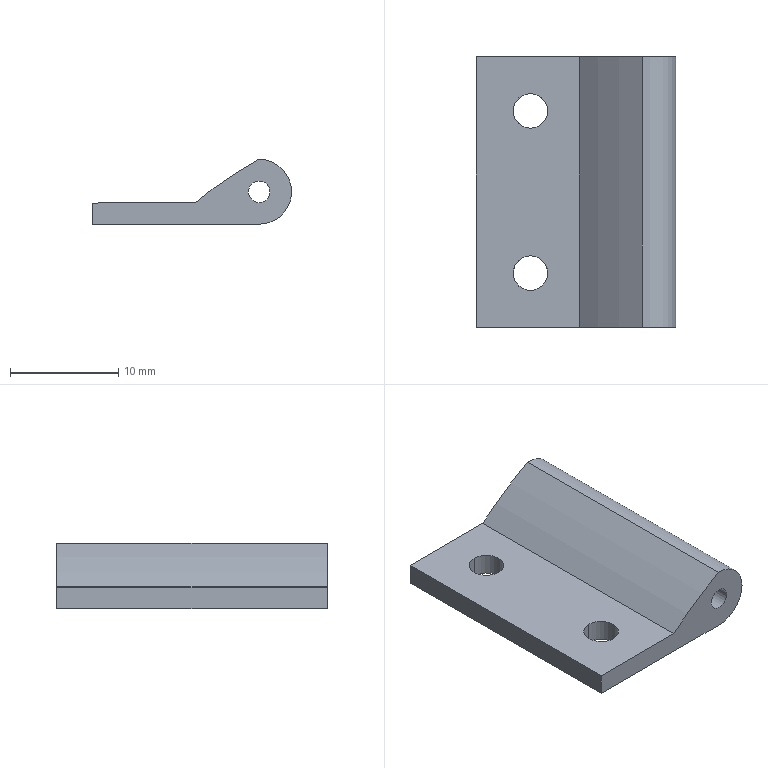Component | SolidWorks | CL201-M6-2-5 | 1 solid | 14 faces | box 18.43 x 25 x 6.04 mm | volume 1333 mm3 | cylinder 8 | plane 5 | spline 1 | commonest cylinder face diameters 3.2 x4 2 x2 6 x2
build123d program:
from build123d import *

# Parameters (mm, degrees)
SKETCH1_R           = 1
BOSS_EXTRUDE1_DEPTH = 25
SKETCH5_R           = 1.6
CUT_EXTRUDE3_DEPTH  = 48


with BuildPart() as part:
    # Sketch1 → Boss-Extrude1 (new body)
    with BuildSketch(Plane.XY):
        with BuildLine():
            Line((-63.314, 21.898), (-47.884, 21.898))
            Line((-47.884, 21.898), (-47.884, 19.898))
            Line((-47.884, 19.898), (-57.401, 19.898))
            add(Edge.make_bspline(
                [(-63.239, 15.899), (-59.863, 17.806), (-57.401, 19.898)],
                knots=[0, 0, 0, 0.7645, 0.7645, 0.7645], degree=2))
            ThreePointArc((-63.239, 15.899), (-66.314, 18.86), (-63.314, 21.898))
        make_face()
        with Locations((-63.314, 18.898)):
            Circle(SKETCH1_R, mode=Mode.SUBTRACT)
    extrude(amount=BOSS_EXTRUDE1_DEPTH)

    # Sketch5 → Cut-Extrude3 (cut)
    with BuildSketch(Plane.XZ.offset(-19.898)):
        with Locations(Location((-52.884, 20, 0), (0, 0, 270))):
            Circle(SKETCH5_R)
        with Locations(Location((-52.884, 5, 0), (0, 0, 270))):
            Circle(SKETCH5_R)
    extrude(amount=-CUT_EXTRUDE3_DEPTH, mode=Mode.SUBTRACT)


solid = part.part

# Placed as in the assembly
solid = solid.moved(Location((248.38, 1902.96, -163.788), (90, 0, -179.857)))
STEP:
#1=CARTESIAN_POINT('',(11.863,74.66,-7.305));
#2=VERTEX_POINT('',#1);
#3=CARTESIAN_POINT('',(11.863,74.786,-7.305));
#4=VERTEX_POINT('',#3);
#5=CARTESIAN_POINT('',(11.863,74.723,-7.305));
#6=DIRECTION('',(-0.002502,-0.,1.));
#7=DIRECTION('',(0.,1.,0.));
#8=AXIS2_PLACEMENT_3D('',#5,#6,#7);
#9=CIRCLE('',#8,0.06299);
#10=EDGE_CURVE('',#2,#4,#9,.T.);
#11=ORIENTED_EDGE('',*,*,#10,.F.);
#12=CARTESIAN_POINT('',(11.863,74.66,-7.227));
#13=VERTEX_POINT('',#12);
#14=CARTESIAN_POINT('',(11.867,74.66,-9.116));
#15=DIRECTION('',(-0.002502,-0.,1.));
#16=VECTOR('',#15,39.37);
#17=LINE('',#14,#16);
#18=EDGE_CURVE('',#2,#13,#17,.T.);
#19=ORIENTED_EDGE('',*,*,#18,.T.);
#20=CARTESIAN_POINT('',(11.863,74.786,-7.227));
#21=VERTEX_POINT('',#20);
#22=CARTESIAN_POINT('',(11.863,74.723,-7.227));
#23=DIRECTION('',(-0.002502,-0.,1.));
#24=DIRECTION('',(0.,1.,0.));
#25=AXIS2_PLACEMENT_3D('',#22,#23,#24);
#26=CIRCLE('',#25,0.06299);
#27=EDGE_CURVE('',#13,#21,#26,.T.);
#28=ORIENTED_EDGE('',*,*,#27,.T.);
#29=CARTESIAN_POINT('',(11.867,74.786,-9.116));
#30=DIRECTION('',(-0.002502,-0.,1.));
#31=VECTOR('',#30,39.37);
#32=LINE('',#29,#31);
#33=EDGE_CURVE('',#4,#21,#32,.T.);
#34=ORIENTED_EDGE('',*,*,#33,.F.);
#35=EDGE_LOOP('',(#11,#19,#28,#34));
#36=FACE_OUTER_BOUND('',#35,.T.);
#37=CARTESIAN_POINT('',(11.867,74.723,-9.116));
#38=DIRECTION('',(-0.002502,-0.,1.));
#39=DIRECTION('',(0.,1.,0.));
#40=AXIS2_PLACEMENT_3D('',#37,#38,#39);
#41=CYLINDRICAL_SURFACE('',#40,0.06299);
#42=ADVANCED_FACE('',(#36),#41,.F.);
#43=CARTESIAN_POINT('',(11.863,74.069,-7.305));
#44=VERTEX_POINT('',#43);
#45=CARTESIAN_POINT('',(11.863,74.195,-7.305));
#46=VERTEX_POINT('',#45);
#47=CARTESIAN_POINT('',(11.863,74.132,-7.305));
#48=DIRECTION('',(-0.002502,-0.,1.));
#49=DIRECTION('',(0.,1.,0.));
#50=AXIS2_PLACEMENT_3D('',#47,#48,#49);
#51=CIRCLE('',#50,0.06299);
#52=EDGE_CURVE('',#44,#46,#51,.T.);
#53=ORIENTED_EDGE('',*,*,#52,.F.);
#54=CARTESIAN_POINT('',(11.863,74.069,-7.227));
#55=VERTEX_POINT('',#54);
#56=CARTESIAN_POINT('',(11.867,74.069,-9.116));
#57=DIRECTION('',(-0.002502,-0.,1.));
#58=VECTOR('',#57,39.37);
#59=LINE('',#56,#58);
#60=EDGE_CURVE('',#44,#55,#59,.T.);
#61=ORIENTED_EDGE('',*,*,#60,.T.);
#62=CARTESIAN_POINT('',(11.863,74.195,-7.227));
#63=VERTEX_POINT('',#62);
#64=CARTESIAN_POINT('',(11.863,74.132,-7.227));
#65=DIRECTION('',(-0.002502,-0.,1.));
#66=DIRECTION('',(0.,1.,0.));
#67=AXIS2_PLACEMENT_3D('',#64,#65,#66);
#68=CIRCLE('',#67,0.06299);
#69=EDGE_CURVE('',#55,#63,#68,.T.);
#70=ORIENTED_EDGE('',*,*,#69,.T.);
#71=CARTESIAN_POINT('',(11.867,74.195,-9.116));
#72=DIRECTION('',(-0.002502,-0.,1.));
#73=VECTOR('',#72,39.37);
#74=LINE('',#71,#73);
#75=EDGE_CURVE('',#46,#63,#74,.T.);
#76=ORIENTED_EDGE('',*,*,#75,.F.);
#77=EDGE_LOOP('',(#53,#61,#70,#76));
#78=FACE_OUTER_BOUND('',#77,.T.);
#79=CARTESIAN_POINT('',(11.867,74.132,-9.116));
#80=DIRECTION('',(-0.002502,-0.,1.));
#81=DIRECTION('',(0.,1.,0.));
#82=AXIS2_PLACEMENT_3D('',#79,#80,#81);
#83=CYLINDRICAL_SURFACE('',#82,0.06299);
#84=ADVANCED_FACE('',(#78),#83,.F.);
#85=CARTESIAN_POINT('',(12.313,73.935,-7.186));
#86=VERTEX_POINT('',#85);
#87=CARTESIAN_POINT('',(12.234,73.935,-7.186));
#88=VERTEX_POINT('',#87);
#89=CARTESIAN_POINT('',(12.273,73.935,-7.186));
#90=DIRECTION('',(0.,-1.,-0.));
#91=DIRECTION('',(-1.,0.,-0.002502));
#92=AXIS2_PLACEMENT_3D('',#89,#90,#91);
#93=CIRCLE('',#92,0.03937);
#94=EDGE_CURVE('',#86,#88,#93,.T.);
#95=ORIENTED_EDGE('',*,*,#94,.T.);
#96=CARTESIAN_POINT('',(12.234,74.92,-7.186));
#97=VERTEX_POINT('',#96);
#98=CARTESIAN_POINT('',(12.234,73.935,-7.186));
#99=DIRECTION('',(-0.,1.,0.));
#100=VECTOR('',#99,39.37);
#101=LINE('',#98,#100);
#102=EDGE_CURVE('',#88,#97,#101,.T.);
#103=ORIENTED_EDGE('',*,*,#102,.T.);
#104=CARTESIAN_POINT('',(12.313,74.92,-7.186));
#105=VERTEX_POINT('',#104);
#106=CARTESIAN_POINT('',(12.273,74.92,-7.186));
#107=DIRECTION('',(0.,-1.,-0.));
#108=DIRECTION('',(-1.,0.,-0.002502));
#109=AXIS2_PLACEMENT_3D('',#106,#107,#108);
#110=CIRCLE('',#109,0.03937);
#111=EDGE_CURVE('',#105,#97,#110,.T.);
#112=ORIENTED_EDGE('',*,*,#111,.F.);
#113=CARTESIAN_POINT('',(12.313,73.935,-7.186));
#114=DIRECTION('',(-0.,1.,0.));
#115=VECTOR('',#114,39.37);
#116=LINE('',#113,#115);
#117=EDGE_CURVE('',#86,#105,#116,.T.);
#118=ORIENTED_EDGE('',*,*,#117,.F.);
#119=EDGE_LOOP('',(#95,#103,#112,#118));
#120=FACE_OUTER_BOUND('',#119,.T.);
#121=CARTESIAN_POINT('',(12.273,73.935,-7.186));
#122=DIRECTION('',(-0.,1.,0.));
#123=DIRECTION('',(1.,0.,0.002502));
#124=AXIS2_PLACEMENT_3D('',#121,#122,#123);
#125=CYLINDRICAL_SURFACE('',#124,0.03937);
#126=ADVANCED_FACE('',(#120),#125,.F.);
#127=CARTESIAN_POINT('',(12.391,73.935,-7.186));
#128=VERTEX_POINT('',#127);
#129=CARTESIAN_POINT('',(12.27,73.935,-7.068));
#130=VERTEX_POINT('',#129);
#131=CARTESIAN_POINT('',(12.273,73.935,-7.186));
#132=DIRECTION('',(0.,-1.,-0.));
#133=DIRECTION('',(-1.,0.,-0.002502));
#134=AXIS2_PLACEMENT_3D('',#131,#132,#133);
#135=CIRCLE('',#134,0.1181);
#136=EDGE_CURVE('',#128,#130,#135,.T.);
#137=ORIENTED_EDGE('',*,*,#136,.F.);
#138=CARTESIAN_POINT('',(12.391,74.92,-7.186));
#139=VERTEX_POINT('',#138);
#140=CARTESIAN_POINT('',(12.391,73.935,-7.186));
#141=DIRECTION('',(-0.,1.,0.));
#142=VECTOR('',#141,39.37);
#143=LINE('',#140,#142);
#144=EDGE_CURVE('',#128,#139,#143,.T.);
#145=ORIENTED_EDGE('',*,*,#144,.T.);
#146=CARTESIAN_POINT('',(12.27,74.92,-7.068));
#147=VERTEX_POINT('',#146);
#148=CARTESIAN_POINT('',(12.273,74.92,-7.186));
#149=DIRECTION('',(0.,-1.,-0.));
#150=DIRECTION('',(-1.,0.,-0.002502));
#151=AXIS2_PLACEMENT_3D('',#148,#149,#150);
#152=CIRCLE('',#151,0.1181);
#153=EDGE_CURVE('',#139,#147,#152,.T.);
#154=ORIENTED_EDGE('',*,*,#153,.T.);
#155=CARTESIAN_POINT('',(12.27,73.935,-7.068));
#156=DIRECTION('',(-0.,1.,0.));
#157=VECTOR('',#156,39.37);
#158=LINE('',#155,#157);
#159=EDGE_CURVE('',#130,#147,#158,.T.);
#160=ORIENTED_EDGE('',*,*,#159,.F.);
#161=EDGE_LOOP('',(#137,#145,#154,#160));
#162=FACE_OUTER_BOUND('',#161,.T.);
#163=CARTESIAN_POINT('',(12.273,73.935,-7.186));
#164=DIRECTION('',(-0.,1.,0.));
#165=DIRECTION('',(1.,0.,0.002502));
#166=AXIS2_PLACEMENT_3D('',#163,#164,#165);
#167=CYLINDRICAL_SURFACE('',#166,0.1181);
#168=ADVANCED_FACE('',(#162),#167,.T.);
#169=CARTESIAN_POINT('',(12.041,73.935,-7.226));
#170=VERTEX_POINT('',#169);
#171=CARTESIAN_POINT('',(12.27,73.935,-7.068));
#172=CARTESIAN_POINT('',(12.137,73.935,-7.143));
#173=CARTESIAN_POINT('',(12.041,73.935,-7.226));
#174=B_SPLINE_CURVE_WITH_KNOTS('',2,(#171,#172,#173),.UNSPECIFIED.,.F.,.F.,(3,3),(0.,0.7645),.UNSPECIFIED.);
#175=EDGE_CURVE('',#130,#170,#174,.T.);
#176=ORIENTED_EDGE('',*,*,#175,.T.);
#177=CARTESIAN_POINT('',(11.666,73.935,-7.227));
#178=VERTEX_POINT('',#177);
#179=CARTESIAN_POINT('',(12.041,73.935,-7.226));
#180=DIRECTION('',(-1.,-0.,-0.002502));
#181=VECTOR('',#180,39.37);
#182=LINE('',#179,#181);
#183=EDGE_CURVE('',#170,#178,#182,.T.);
#184=ORIENTED_EDGE('',*,*,#183,.T.);
#185=CARTESIAN_POINT('',(11.666,73.935,-7.306));
#186=VERTEX_POINT('',#185);
#187=CARTESIAN_POINT('',(11.666,73.935,-7.306));
#188=DIRECTION('',(0.002502,0.,-1.));
#189=VECTOR('',#188,39.37);
#190=LINE('',#187,#189);
#191=EDGE_CURVE('',#178,#186,#190,.T.);
#192=ORIENTED_EDGE('',*,*,#191,.T.);
#193=CARTESIAN_POINT('',(12.274,73.935,-7.304));
#194=VERTEX_POINT('',#193);
#195=CARTESIAN_POINT('',(12.274,73.935,-7.304));
#196=DIRECTION('',(1.,0.,0.002502));
#197=VECTOR('',#196,39.37);
#198=LINE('',#195,#197);
#199=EDGE_CURVE('',#186,#194,#198,.T.);
#200=ORIENTED_EDGE('',*,*,#199,.T.);
#201=CARTESIAN_POINT('',(12.273,73.935,-7.186));
#202=DIRECTION('',(0.,-1.,-0.));
#203=DIRECTION('',(-1.,0.,-0.002502));
#204=AXIS2_PLACEMENT_3D('',#201,#202,#203);
#205=CIRCLE('',#204,0.1181);
#206=EDGE_CURVE('',#194,#128,#205,.T.);
#207=ORIENTED_EDGE('',*,*,#206,.T.);
#208=ORIENTED_EDGE('',*,*,#136,.T.);
#209=EDGE_LOOP('',(#176,#184,#192,#200,#207,#208));
#210=FACE_OUTER_BOUND('',#209,.T.);
#211=ORIENTED_EDGE('',*,*,#94,.F.);
#212=CARTESIAN_POINT('',(12.273,73.935,-7.186));
#213=DIRECTION('',(0.,-1.,-0.));
#214=DIRECTION('',(-1.,0.,-0.002502));
#215=AXIS2_PLACEMENT_3D('',#212,#213,#214);
#216=CIRCLE('',#215,0.03937);
#217=EDGE_CURVE('',#88,#86,#216,.T.);
#218=ORIENTED_EDGE('',*,*,#217,.F.);
#219=EDGE_LOOP('',(#211,#218));
#220=FACE_BOUND('',#219,.T.);
#221=CARTESIAN_POINT('',(12.146,73.935,-7.145));
#222=DIRECTION('',(-0.,1.,0.));
#223=DIRECTION('',(1.,0.,0.002502));
#224=AXIS2_PLACEMENT_3D('',#221,#222,#223);
#225=PLANE('',#224);
#226=ADVANCED_FACE('',(#210,#220),#225,.F.);
#227=CARTESIAN_POINT('',(12.041,74.92,-7.226));
#228=VERTEX_POINT('',#227);
#229=CARTESIAN_POINT('',(12.27,74.92,-7.068));
#230=CARTESIAN_POINT('',(12.137,74.92,-7.143));
#231=CARTESIAN_POINT('',(12.041,74.92,-7.226));
#232=B_SPLINE_CURVE_WITH_KNOTS('',2,(#229,#230,#231),.UNSPECIFIED.,.F.,.F.,(3,3),(0.,0.7645),.UNSPECIFIED.);
#233=EDGE_CURVE('',#147,#228,#232,.T.);
#234=ORIENTED_EDGE('',*,*,#233,.F.);
#235=ORIENTED_EDGE('',*,*,#153,.F.);
#236=CARTESIAN_POINT('',(12.274,74.92,-7.304));
#237=VERTEX_POINT('',#236);
#238=CARTESIAN_POINT('',(12.273,74.92,-7.186));
#239=DIRECTION('',(0.,-1.,-0.));
#240=DIRECTION('',(-1.,0.,-0.002502));
#241=AXIS2_PLACEMENT_3D('',#238,#239,#240);
#242=CIRCLE('',#241,0.1181);
#243=EDGE_CURVE('',#237,#139,#242,.T.);
#244=ORIENTED_EDGE('',*,*,#243,.F.);
#245=CARTESIAN_POINT('',(11.666,74.92,-7.306));
#246=VERTEX_POINT('',#245);
#247=CARTESIAN_POINT('',(12.274,74.92,-7.304));
#248=DIRECTION('',(1.,0.,0.002502));
#249=VECTOR('',#248,39.37);
#250=LINE('',#247,#249);
#251=EDGE_CURVE('',#246,#237,#250,.T.);
#252=ORIENTED_EDGE('',*,*,#251,.F.);
#253=CARTESIAN_POINT('',(11.666,74.92,-7.227));
#254=VERTEX_POINT('',#253);
#255=CARTESIAN_POINT('',(11.666,74.92,-7.306));
#256=DIRECTION('',(0.002502,0.,-1.));
#257=VECTOR('',#256,39.37);
#258=LINE('',#255,#257);
#259=EDGE_CURVE('',#254,#246,#258,.T.);
#260=ORIENTED_EDGE('',*,*,#259,.F.);
#261=CARTESIAN_POINT('',(12.041,74.92,-7.226));
#262=DIRECTION('',(-1.,-0.,-0.002502));
#263=VECTOR('',#262,39.37);
#264=LINE('',#261,#263);
#265=EDGE_CURVE('',#228,#254,#264,.T.);
#266=ORIENTED_EDGE('',*,*,#265,.F.);
#267=EDGE_LOOP('',(#234,#235,#244,#252,#260,#266));
#268=FACE_OUTER_BOUND('',#267,.T.);
#269=ORIENTED_EDGE('',*,*,#111,.T.);
#270=CARTESIAN_POINT('',(12.273,74.92,-7.186));
#271=DIRECTION('',(0.,-1.,-0.));
#272=DIRECTION('',(-1.,0.,-0.002502));
#273=AXIS2_PLACEMENT_3D('',#270,#271,#272);
#274=CIRCLE('',#273,0.03937);
#275=EDGE_CURVE('',#97,#105,#274,.T.);
#276=ORIENTED_EDGE('',*,*,#275,.T.);
#277=EDGE_LOOP('',(#269,#276));
#278=FACE_BOUND('',#277,.T.);
#279=CARTESIAN_POINT('',(12.146,74.92,-7.145));
#280=DIRECTION('',(-0.,1.,0.));
#281=DIRECTION('',(1.,0.,0.002502));
#282=AXIS2_PLACEMENT_3D('',#279,#280,#281);
#283=PLANE('',#282);
#284=ADVANCED_FACE('',(#268,#278),#283,.T.);
#285=ORIENTED_EDGE('',*,*,#233,.T.);
#286=CARTESIAN_POINT('',(12.041,73.935,-7.226));
#287=DIRECTION('',(-0.,1.,0.));
#288=VECTOR('',#287,39.37);
#289=LINE('',#286,#288);
#290=EDGE_CURVE('',#170,#228,#289,.T.);
#291=ORIENTED_EDGE('',*,*,#290,.F.);
#292=ORIENTED_EDGE('',*,*,#175,.F.);
#293=ORIENTED_EDGE('',*,*,#159,.T.);
#294=EDGE_LOOP('',(#285,#291,#292,#293));
#295=FACE_OUTER_BOUND('',#294,.T.);
#296=CARTESIAN_POINT('',(12.27,73.935,-7.068));
#297=CARTESIAN_POINT('',(12.27,74.92,-7.068));
#298=CARTESIAN_POINT('',(12.137,73.935,-7.143));
#299=CARTESIAN_POINT('',(12.137,74.92,-7.143));
#300=CARTESIAN_POINT('',(12.041,73.935,-7.226));
#301=CARTESIAN_POINT('',(12.041,74.92,-7.226));
#302=B_SPLINE_SURFACE_WITH_KNOTS('',2,1,((#296,#297),(#298,#299),(#300,#301)),.UNSPECIFIED.,.F.,.F.,.F.,(3,3),(2,2),(0.,0.7645),(0.,1.),.UNSPECIFIED.);
#303=ADVANCED_FACE('',(#295),#302,.F.);
#304=CARTESIAN_POINT('',(11.863,74.723,-7.227));
#305=DIRECTION('',(-0.002502,-0.,1.));
#306=DIRECTION('',(0.,1.,0.));
#307=AXIS2_PLACEMENT_3D('',#304,#305,#306);
#308=CIRCLE('',#307,0.06299);
#309=EDGE_CURVE('',#21,#13,#308,.T.);
#310=ORIENTED_EDGE('',*,*,#309,.F.);
#311=ORIENTED_EDGE('',*,*,#27,.F.);
#312=EDGE_LOOP('',(#310,#311));
#313=FACE_BOUND('',#312,.T.);
#314=CARTESIAN_POINT('',(11.863,74.132,-7.227));
#315=DIRECTION('',(-0.002502,-0.,1.));
#316=DIRECTION('',(0.,1.,0.));
#317=AXIS2_PLACEMENT_3D('',#314,#315,#316);
#318=CIRCLE('',#317,0.06299);
#319=EDGE_CURVE('',#63,#55,#318,.T.);
#320=ORIENTED_EDGE('',*,*,#319,.F.);
#321=ORIENTED_EDGE('',*,*,#69,.F.);
#322=EDGE_LOOP('',(#320,#321));
#323=FACE_BOUND('',#322,.T.);
#324=ORIENTED_EDGE('',*,*,#265,.T.);
#325=CARTESIAN_POINT('',(11.666,73.935,-7.227));
#326=DIRECTION('',(-0.,1.,0.));
#327=VECTOR('',#326,39.37);
#328=LINE('',#325,#327);
#329=EDGE_CURVE('',#178,#254,#328,.T.);
#330=ORIENTED_EDGE('',*,*,#329,.F.);
#331=ORIENTED_EDGE('',*,*,#183,.F.);
#332=ORIENTED_EDGE('',*,*,#290,.T.);
#333=EDGE_LOOP('',(#324,#330,#331,#332));
#334=FACE_OUTER_BOUND('',#333,.T.);
#335=CARTESIAN_POINT('',(12.041,73.935,-7.226));
#336=DIRECTION('',(0.002502,0.,-1.));
#337=DIRECTION('',(0.,-1.,-0.));
#338=AXIS2_PLACEMENT_3D('',#335,#336,#337);
#339=PLANE('',#338);
#340=ADVANCED_FACE('',(#313,#323,#334),#339,.F.);
#341=ORIENTED_EDGE('',*,*,#259,.T.);
#342=CARTESIAN_POINT('',(11.666,73.935,-7.306));
#343=DIRECTION('',(-0.,1.,0.));
#344=VECTOR('',#343,39.37);
#345=LINE('',#342,#344);
#346=EDGE_CURVE('',#186,#246,#345,.T.);
#347=ORIENTED_EDGE('',*,*,#346,.F.);
#348=ORIENTED_EDGE('',*,*,#191,.F.);
#349=ORIENTED_EDGE('',*,*,#329,.T.);
#350=EDGE_LOOP('',(#341,#347,#348,#349));
#351=FACE_OUTER_BOUND('',#350,.T.);
#352=CARTESIAN_POINT('',(11.666,73.935,-7.306));
#353=DIRECTION('',(1.,0.,0.002502));
#354=DIRECTION('',(0.,-1.,-0.));
#355=AXIS2_PLACEMENT_3D('',#352,#353,#354);
#356=PLANE('',#355);
#357=ADVANCED_FACE('',(#351),#356,.F.);
#358=CARTESIAN_POINT('',(11.863,74.723,-7.305));
#359=DIRECTION('',(-0.002502,-0.,1.));
#360=DIRECTION('',(0.,1.,0.));
#361=AXIS2_PLACEMENT_3D('',#358,#359,#360);
#362=CIRCLE('',#361,0.06299);
#363=EDGE_CURVE('',#4,#2,#362,.T.);
#364=ORIENTED_EDGE('',*,*,#363,.T.);
#365=ORIENTED_EDGE('',*,*,#10,.T.);
#366=EDGE_LOOP('',(#364,#365));
#367=FACE_BOUND('',#366,.T.);
#368=CARTESIAN_POINT('',(11.863,74.132,-7.305));
#369=DIRECTION('',(-0.002502,-0.,1.));
#370=DIRECTION('',(0.,1.,0.));
#371=AXIS2_PLACEMENT_3D('',#368,#369,#370);
#372=CIRCLE('',#371,0.06299);
#373=EDGE_CURVE('',#46,#44,#372,.T.);
#374=ORIENTED_EDGE('',*,*,#373,.T.);
#375=ORIENTED_EDGE('',*,*,#52,.T.);
#376=EDGE_LOOP('',(#374,#375));
#377=FACE_BOUND('',#376,.T.);
#378=ORIENTED_EDGE('',*,*,#251,.T.);
#379=CARTESIAN_POINT('',(12.274,73.935,-7.304));
#380=DIRECTION('',(-0.,1.,0.));
#381=VECTOR('',#380,39.37);
#382=LINE('',#379,#381);
#383=EDGE_CURVE('',#194,#237,#382,.T.);
#384=ORIENTED_EDGE('',*,*,#383,.F.);
#385=ORIENTED_EDGE('',*,*,#199,.F.);
#386=ORIENTED_EDGE('',*,*,#346,.T.);
#387=EDGE_LOOP('',(#378,#384,#385,#386));
#388=FACE_OUTER_BOUND('',#387,.T.);
#389=CARTESIAN_POINT('',(12.274,73.935,-7.304));
#390=DIRECTION('',(-0.002502,-0.,1.));
#391=DIRECTION('',(-0.,1.,0.));
#392=AXIS2_PLACEMENT_3D('',#389,#390,#391);
#393=PLANE('',#392);
#394=ADVANCED_FACE('',(#367,#377,#388),#393,.F.);
#395=ORIENTED_EDGE('',*,*,#144,.F.);
#396=ORIENTED_EDGE('',*,*,#206,.F.);
#397=ORIENTED_EDGE('',*,*,#383,.T.);
#398=ORIENTED_EDGE('',*,*,#243,.T.);
#399=EDGE_LOOP('',(#395,#396,#397,#398));
#400=FACE_OUTER_BOUND('',#399,.T.);
#401=CARTESIAN_POINT('',(12.273,73.935,-7.186));
#402=DIRECTION('',(-0.,1.,0.));
#403=DIRECTION('',(1.,0.,0.002502));
#404=AXIS2_PLACEMENT_3D('',#401,#402,#403);
#405=CYLINDRICAL_SURFACE('',#404,0.1181);
#406=ADVANCED_FACE('',(#400),#405,.T.);
#407=ORIENTED_EDGE('',*,*,#102,.F.);
#408=ORIENTED_EDGE('',*,*,#217,.T.);
#409=ORIENTED_EDGE('',*,*,#117,.T.);
#410=ORIENTED_EDGE('',*,*,#275,.F.);
#411=EDGE_LOOP('',(#407,#408,#409,#410));
#412=FACE_OUTER_BOUND('',#411,.T.);
#413=CARTESIAN_POINT('',(12.273,73.935,-7.186));
#414=DIRECTION('',(-0.,1.,0.));
#415=DIRECTION('',(1.,0.,0.002502));
#416=AXIS2_PLACEMENT_3D('',#413,#414,#415);
#417=CYLINDRICAL_SURFACE('',#416,0.03937);
#418=ADVANCED_FACE('',(#412),#417,.F.);
#419=ORIENTED_EDGE('',*,*,#60,.F.);
#420=ORIENTED_EDGE('',*,*,#373,.F.);
#421=ORIENTED_EDGE('',*,*,#75,.T.);
#422=ORIENTED_EDGE('',*,*,#319,.T.);
#423=EDGE_LOOP('',(#419,#420,#421,#422));
#424=FACE_OUTER_BOUND('',#423,.T.);
#425=CARTESIAN_POINT('',(11.867,74.132,-9.116));
#426=DIRECTION('',(-0.002502,-0.,1.));
#427=DIRECTION('',(0.,1.,0.));
#428=AXIS2_PLACEMENT_3D('',#425,#426,#427);
#429=CYLINDRICAL_SURFACE('',#428,0.06299);
#430=ADVANCED_FACE('',(#424),#429,.F.);
#431=ORIENTED_EDGE('',*,*,#18,.F.);
#432=ORIENTED_EDGE('',*,*,#363,.F.);
#433=ORIENTED_EDGE('',*,*,#33,.T.);
#434=ORIENTED_EDGE('',*,*,#309,.T.);
#435=EDGE_LOOP('',(#431,#432,#433,#434));
#436=FACE_OUTER_BOUND('',#435,.T.);
#437=CARTESIAN_POINT('',(11.867,74.723,-9.116));
#438=DIRECTION('',(-0.002502,-0.,1.));
#439=DIRECTION('',(0.,1.,0.));
#440=AXIS2_PLACEMENT_3D('',#437,#438,#439);
#441=CYLINDRICAL_SURFACE('',#440,0.06299);
#442=ADVANCED_FACE('',(#436),#441,.F.);
#443=CLOSED_SHELL('',(#42,#84,#126,#168,#226,#284,#303,#340,#357,#394,#406,#418,#430,#442));
#444=MANIFOLD_SOLID_BREP('',#443);
#445=CARTESIAN_POINT('',(0.,0.,0.));
#446=DIRECTION('',(0.,0.,1.));
#447=DIRECTION('',(1.,0.,0.));
#448=AXIS2_PLACEMENT_3D('',#445,#446,#447);
#449=(LENGTH_UNIT()NAMED_UNIT(*)SI_UNIT($,.METRE.));
#450=LENGTH_MEASURE_WITH_UNIT(LENGTH_MEASURE(0.0254),#449);
#451=DIMENSIONAL_EXPONENTS(1.,0.,0.,0.,0.,0.,0.);
#452=(CONVERSION_BASED_UNIT('',#450)LENGTH_UNIT()NAMED_UNIT(#451));
#453=UNCERTAINTY_MEASURE_WITH_UNIT(LENGTH_MEASURE(0.00001),#452,'','');
#454=(NAMED_UNIT(*)PLANE_ANGLE_UNIT()SI_UNIT($,.RADIAN.));
#455=(NAMED_UNIT(*)SI_UNIT($,.STERADIAN.)SOLID_ANGLE_UNIT());
#456=(GEOMETRIC_REPRESENTATION_CONTEXT(3)GLOBAL_UNCERTAINTY_ASSIGNED_CONTEXT((#453))GLOBAL_UNIT_ASSIGNED_CONTEXT((#452,#454,#455))REPRESENTATION_CONTEXT('',''));
#457=ADVANCED_BREP_SHAPE_REPRESENTATION('',(#444,#448),#456);
#458=COLOUR_RGB('',0.7922,0.8196,0.9333);
#459=FILL_AREA_STYLE_COLOUR('',#458);
#460=FILL_AREA_STYLE('',(#459));
#461=SURFACE_STYLE_FILL_AREA(#460);
#462=SURFACE_SIDE_STYLE('',(#461));
#463=SURFACE_STYLE_USAGE(.BOTH.,#462);
#464=PRESENTATION_STYLE_ASSIGNMENT((#463));
#465=STYLED_ITEM('',(#464),#444);
#466=PRESENTATION_LAYER_ASSIGNMENT('','',(#465));
#467=(LENGTH_UNIT()NAMED_UNIT(*)SI_UNIT($,.METRE.));
#468=LENGTH_MEASURE_WITH_UNIT(LENGTH_MEASURE(0.0254),#467);
#469=DIMENSIONAL_EXPONENTS(1.,0.,0.,0.,0.,0.,0.);
#470=(CONVERSION_BASED_UNIT('',#468)LENGTH_UNIT()NAMED_UNIT(#469));
#471=UNCERTAINTY_MEASURE_WITH_UNIT(LENGTH_MEASURE(0.00001),#470,'','');
#472=(NAMED_UNIT(*)PLANE_ANGLE_UNIT()SI_UNIT($,.RADIAN.));
#473=(NAMED_UNIT(*)SI_UNIT($,.STERADIAN.)SOLID_ANGLE_UNIT());
#474=(GEOMETRIC_REPRESENTATION_CONTEXT(3)GLOBAL_UNCERTAINTY_ASSIGNED_CONTEXT((#471))GLOBAL_UNIT_ASSIGNED_CONTEXT((#470,#472,#473))REPRESENTATION_CONTEXT('',''));
#475=MECHANICAL_DESIGN_GEOMETRIC_PRESENTATION_REPRESENTATION('',(#465),#474);